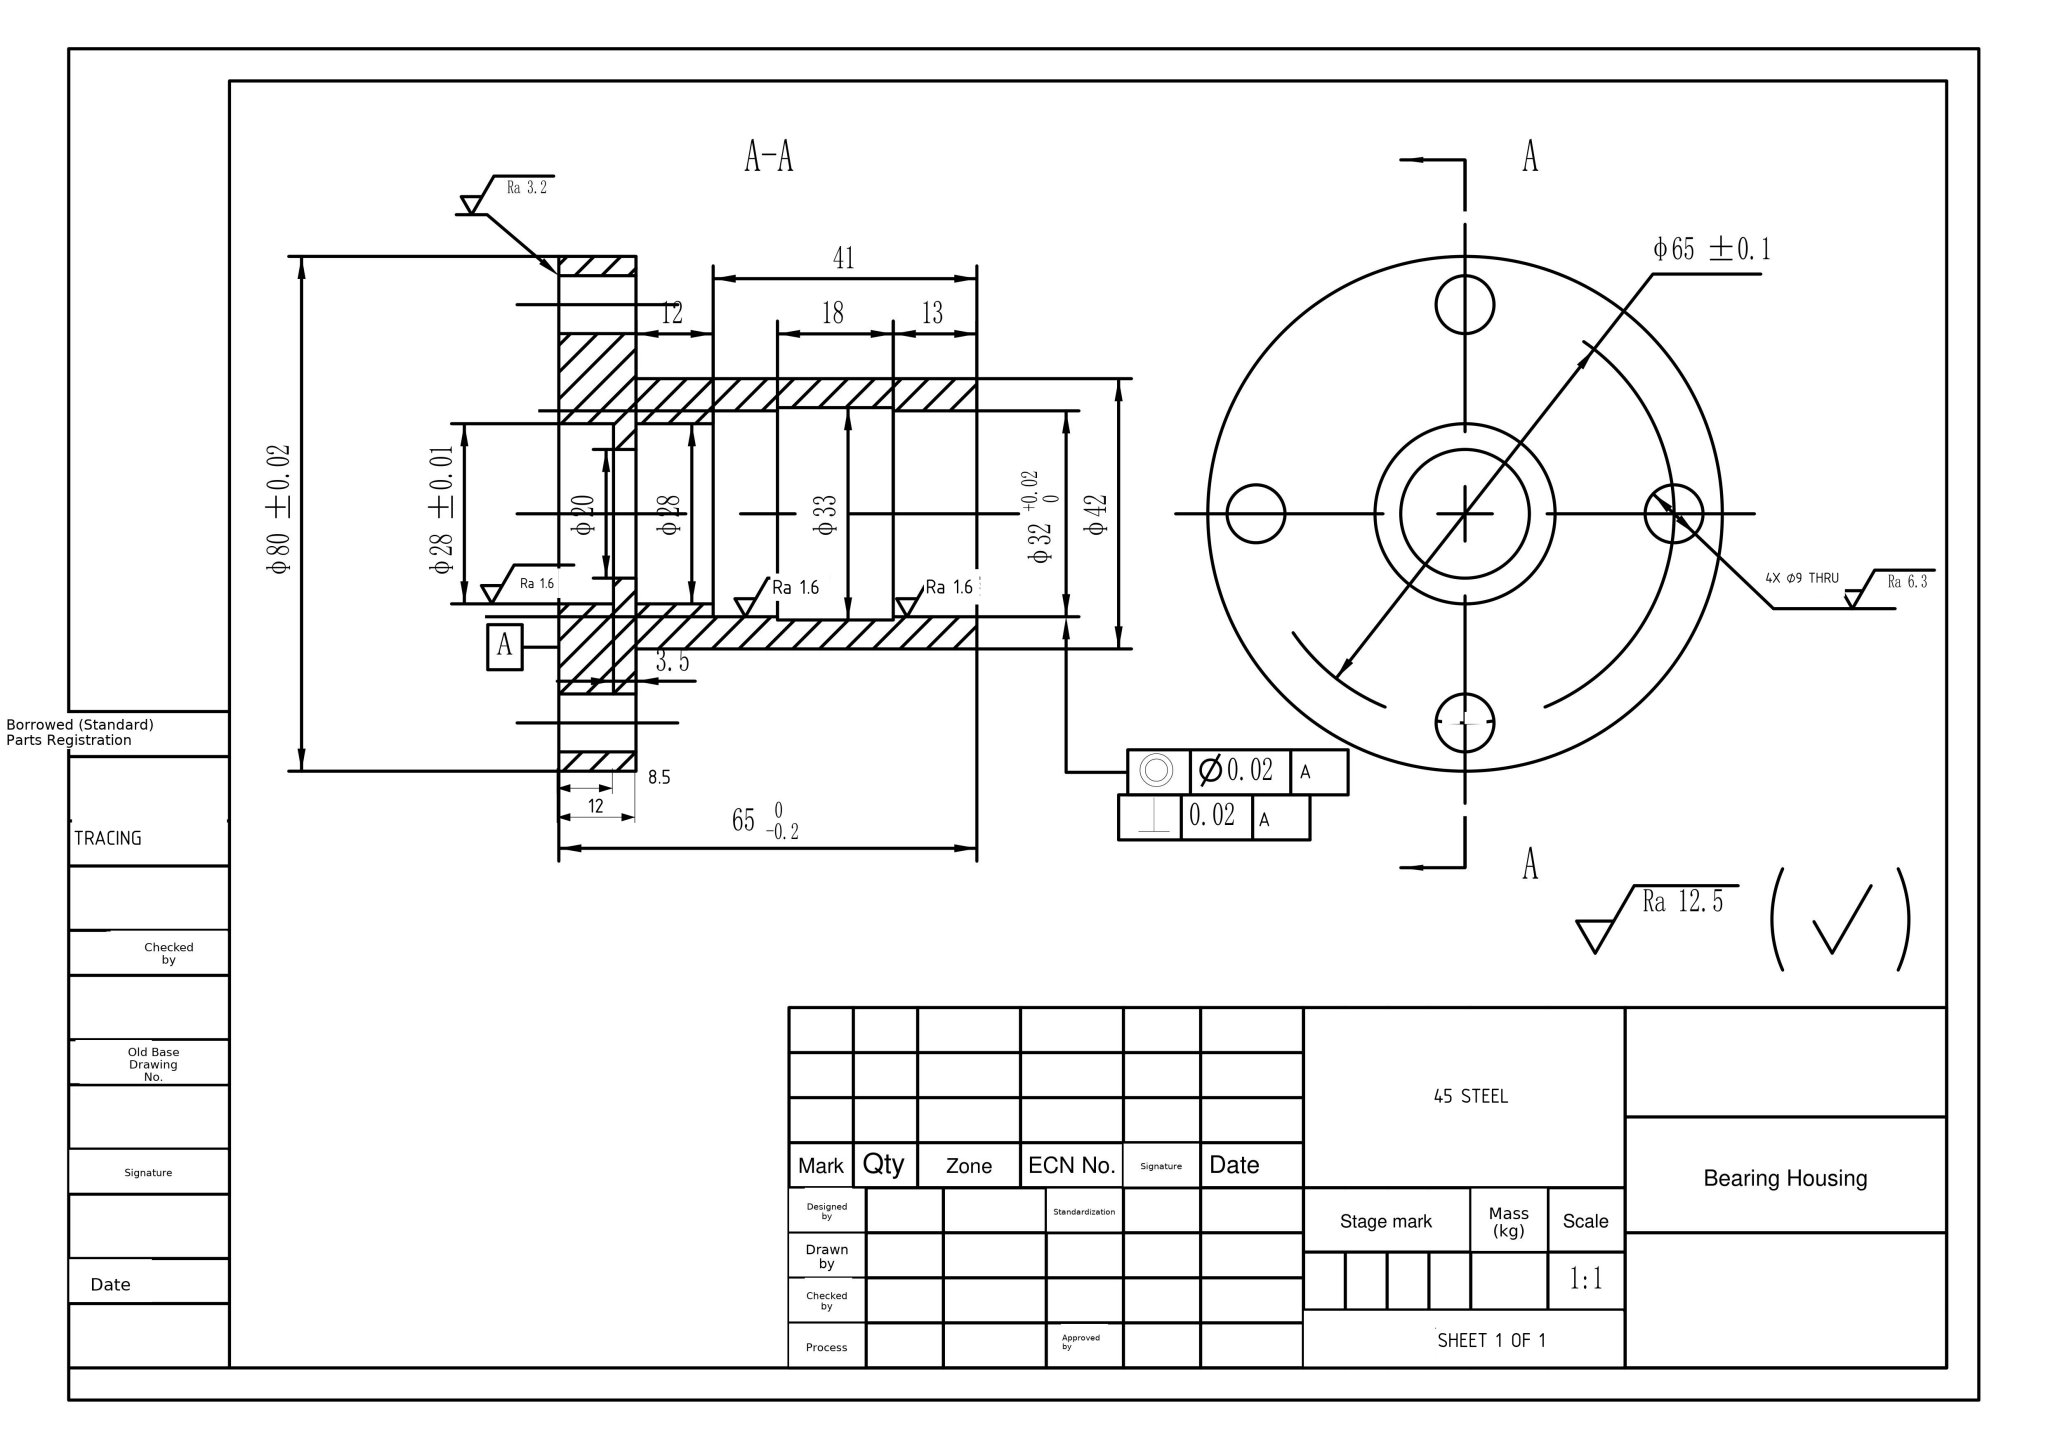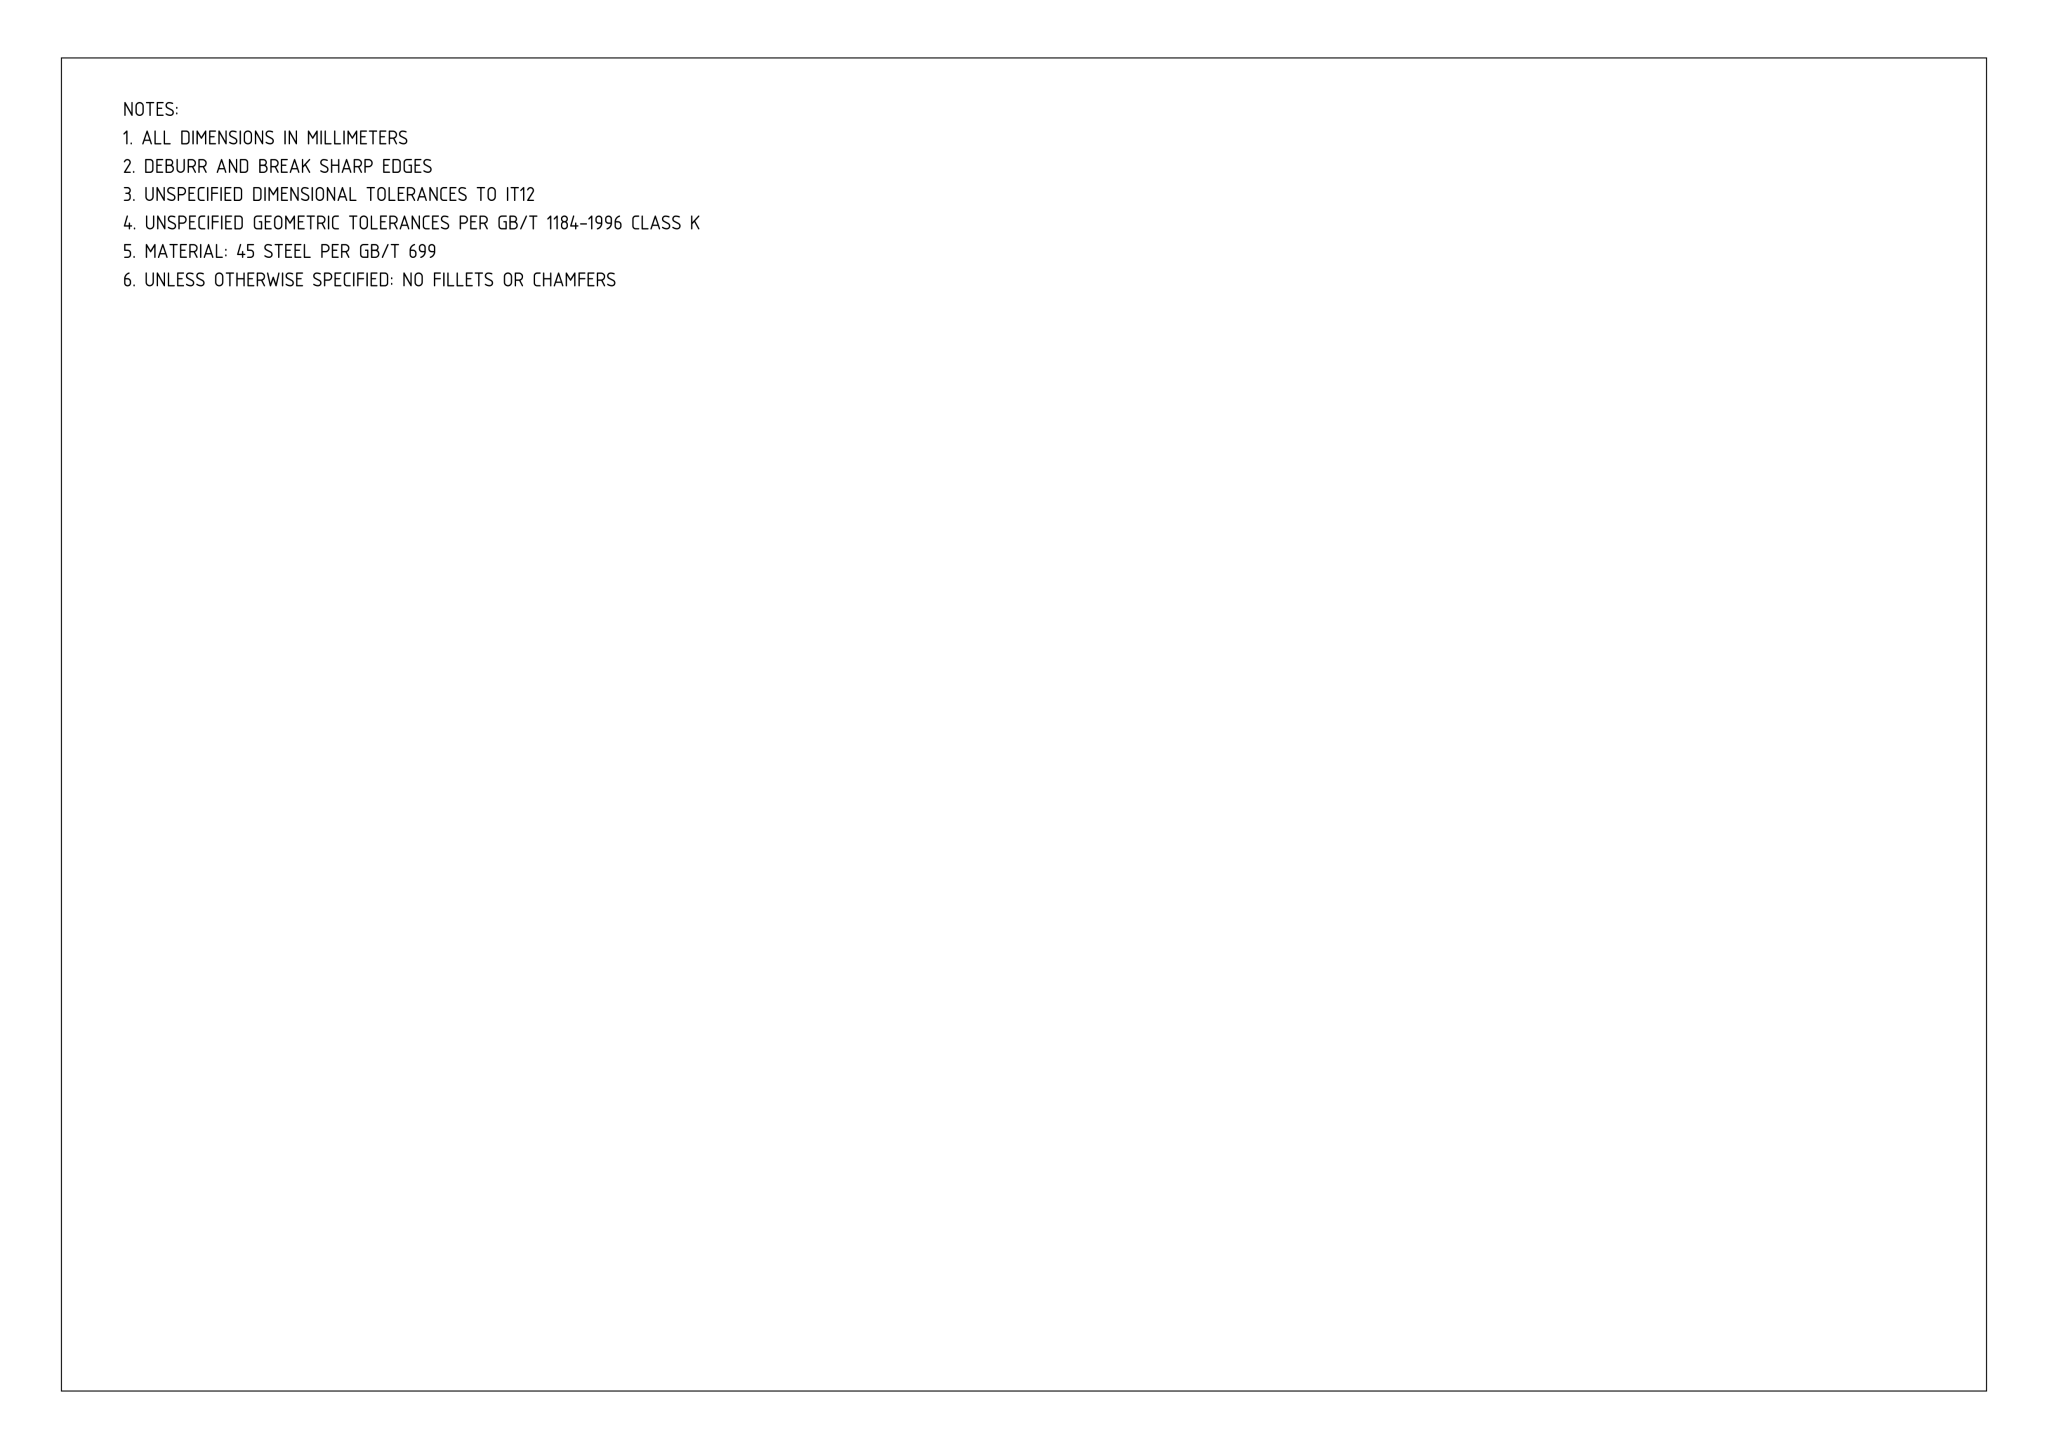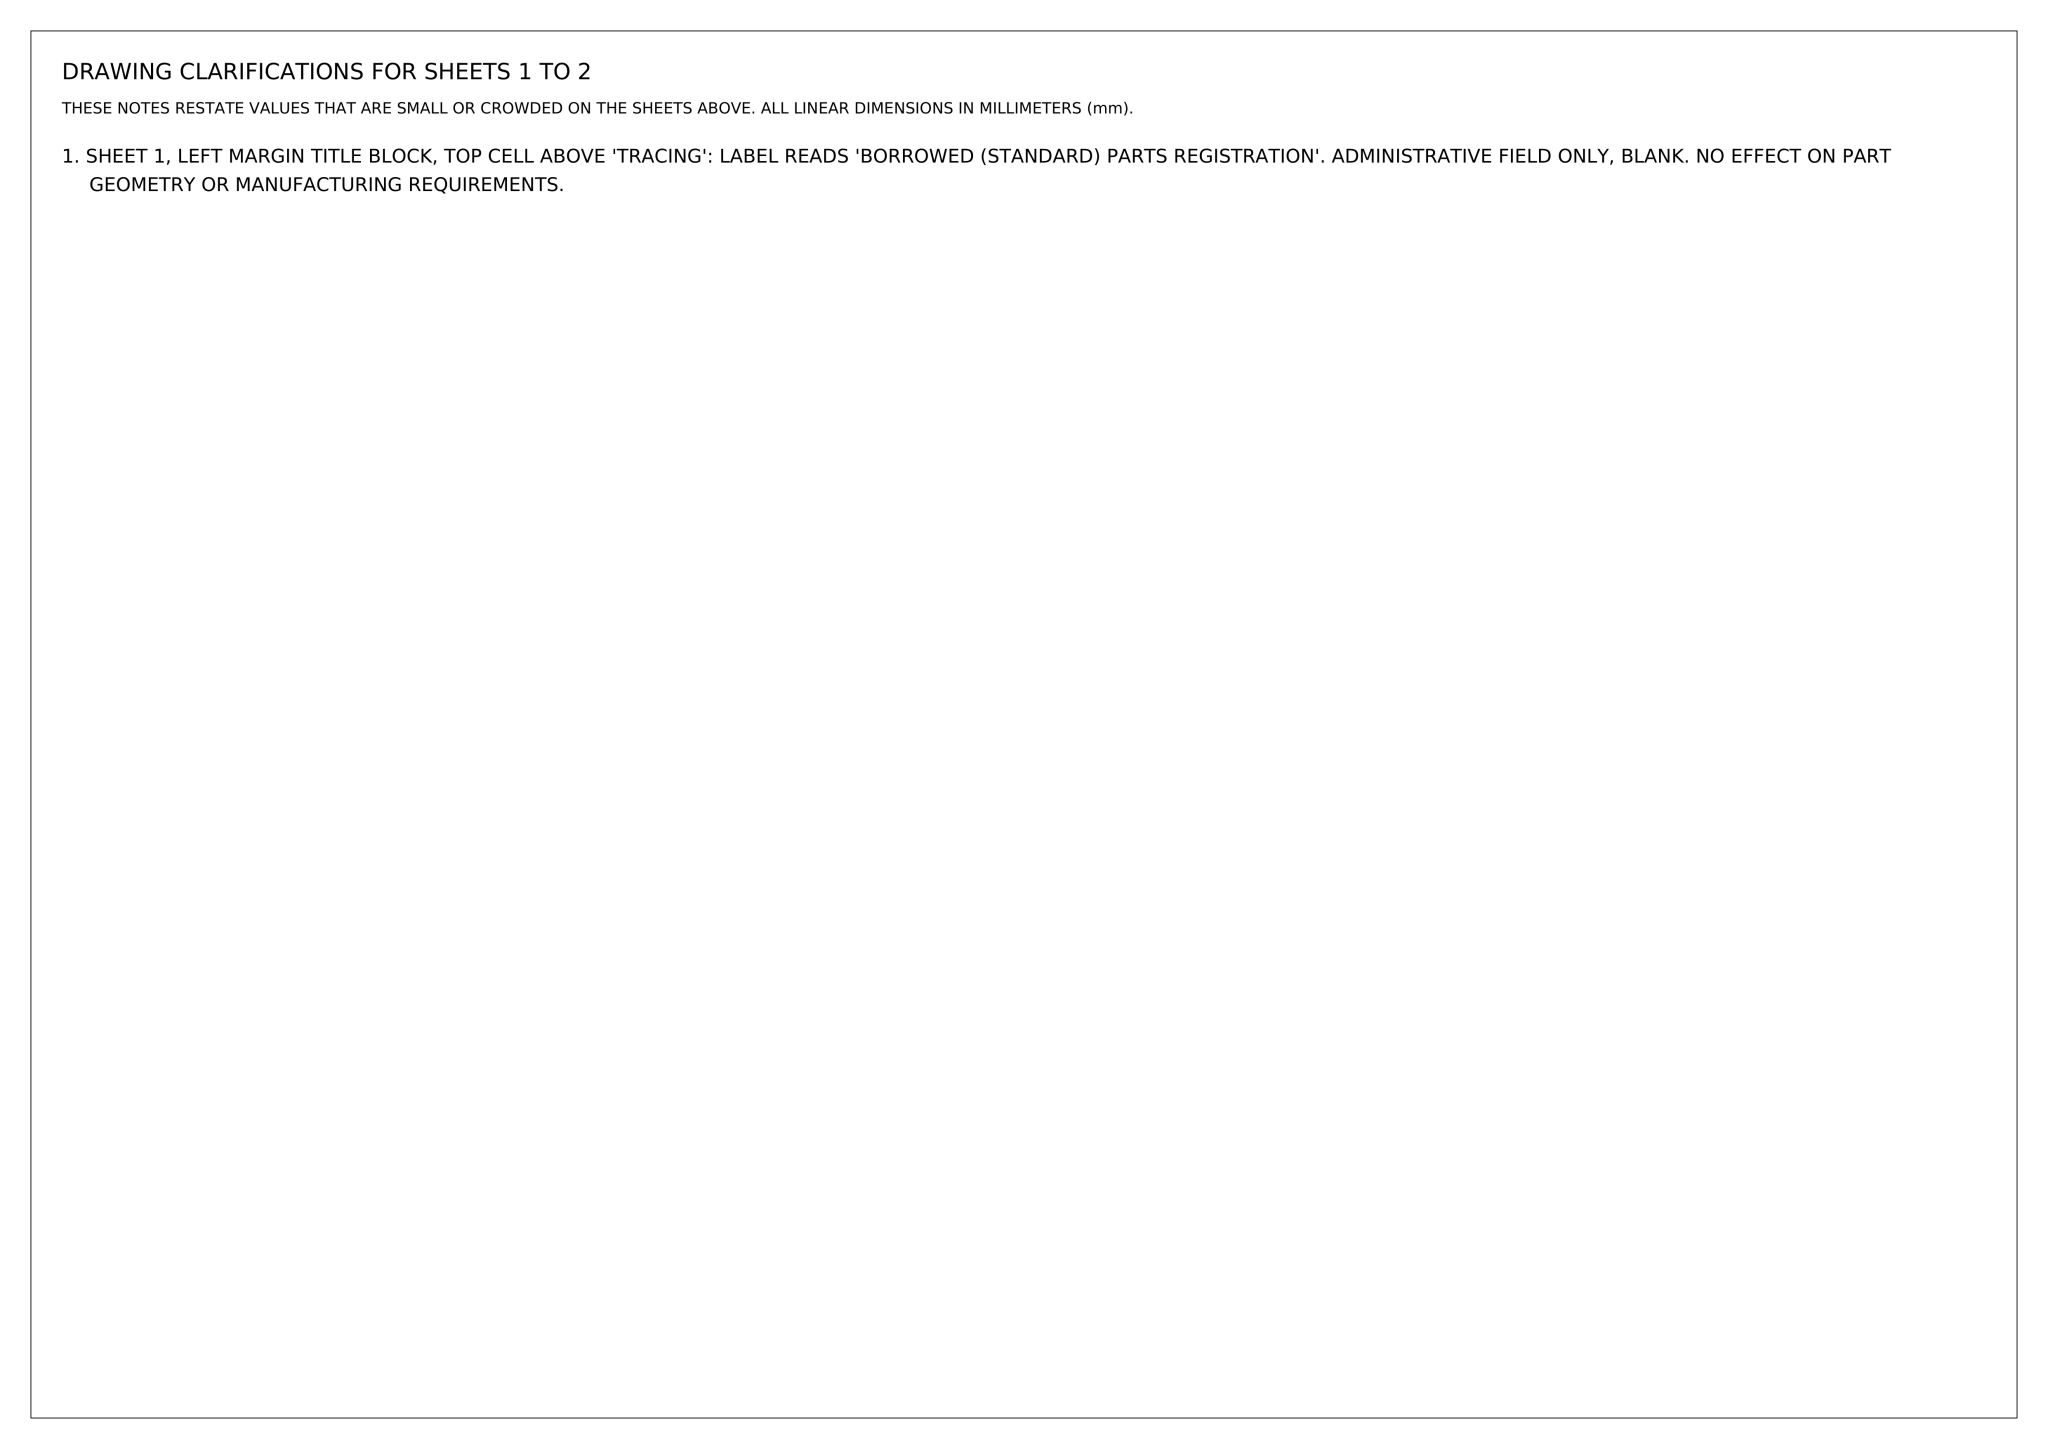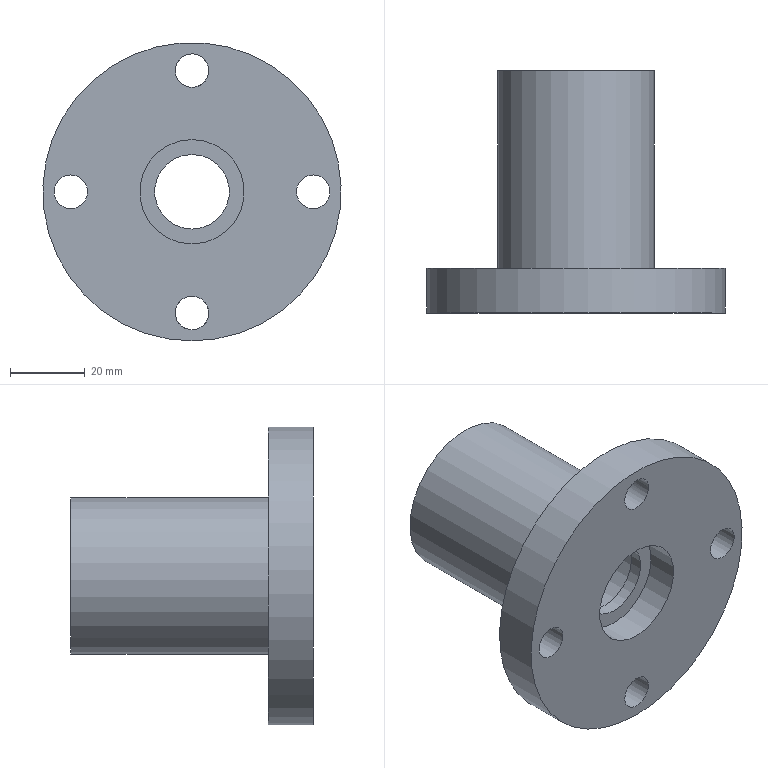Part | NX | mm | 1 solid | 20 faces | box 80 x 65 x 80 mm | volume 83078 mm3 | cylinder 12 | plane 8 | commonest cylinder face diameters 9 x4 28 x2 32 x2 20 x1 33 x1 42 x1 80 x1
STEP:
#1=CARTESIAN_POINT('',(0.,0.,0.));
#2=DIRECTION('',(0.,0.,1.));
#3=DIRECTION('',(1.,0.,0.));
#4=AXIS2_PLACEMENT_3D('',#1,#2,#3);
#5=(LENGTH_UNIT()NAMED_UNIT(*)SI_UNIT(.MILLI.,.METRE.));
#6=UNCERTAINTY_MEASURE_WITH_UNIT(LENGTH_MEASURE(0.00002),#5,'','');
#7=(NAMED_UNIT(*)PLANE_ANGLE_UNIT()SI_UNIT($,.RADIAN.));
#8=PLANE_ANGLE_MEASURE_WITH_UNIT(PLANE_ANGLE_MEASURE(0.01745),#7);
#9=DIMENSIONAL_EXPONENTS(0.,0.,0.,0.,0.,0.,0.);
#10=(CONVERSION_BASED_UNIT('',#8)NAMED_UNIT(#9)PLANE_ANGLE_UNIT());
#11=(NAMED_UNIT(*)SI_UNIT($,.STERADIAN.)SOLID_ANGLE_UNIT());
#12=(GEOMETRIC_REPRESENTATION_CONTEXT(3)GLOBAL_UNCERTAINTY_ASSIGNED_CONTEXT((#6))GLOBAL_UNIT_ASSIGNED_CONTEXT((#5,#10,#11))REPRESENTATION_CONTEXT('',''));
#13=SHAPE_REPRESENTATION('',(#4),#12);
#14=CARTESIAN_POINT('',(32.5,0.,-4.5));
#15=VERTEX_POINT('',#14);
#16=CARTESIAN_POINT('',(32.5,0.,0.));
#17=DIRECTION('',(0.,-1.,0.));
#18=DIRECTION('',(0.,0.,-1.));
#19=AXIS2_PLACEMENT_3D('',#16,#17,#18);
#20=CIRCLE('',#19,4.5);
#21=EDGE_CURVE('',#15,#15,#20,.T.);
#22=ORIENTED_EDGE('',*,*,#21,.F.);
#23=EDGE_LOOP('',(#22));
#24=FACE_BOUND('',#23,.T.);
#25=CARTESIAN_POINT('',(-4.5,0.,-32.5));
#26=VERTEX_POINT('',#25);
#27=CARTESIAN_POINT('',(0.,0.,-32.5));
#28=DIRECTION('',(0.,-1.,0.));
#29=DIRECTION('',(-1.,0.,0.));
#30=AXIS2_PLACEMENT_3D('',#27,#28,#29);
#31=CIRCLE('',#30,4.5);
#32=EDGE_CURVE('',#26,#26,#31,.T.);
#33=ORIENTED_EDGE('',*,*,#32,.F.);
#34=EDGE_LOOP('',(#33));
#35=FACE_BOUND('',#34,.T.);
#36=CARTESIAN_POINT('',(-32.5,0.,4.5));
#37=VERTEX_POINT('',#36);
#38=CARTESIAN_POINT('',(-32.5,0.,0.));
#39=DIRECTION('',(0.,-1.,0.));
#40=DIRECTION('',(0.,0.,1.));
#41=AXIS2_PLACEMENT_3D('',#38,#39,#40);
#42=CIRCLE('',#41,4.5);
#43=EDGE_CURVE('',#37,#37,#42,.T.);
#44=ORIENTED_EDGE('',*,*,#43,.F.);
#45=EDGE_LOOP('',(#44));
#46=FACE_BOUND('',#45,.T.);
#47=CARTESIAN_POINT('',(4.5,0.,32.5));
#48=VERTEX_POINT('',#47);
#49=CARTESIAN_POINT('',(0.,0.,32.5));
#50=DIRECTION('',(0.,-1.,0.));
#51=DIRECTION('',(1.,0.,0.));
#52=AXIS2_PLACEMENT_3D('',#49,#50,#51);
#53=CIRCLE('',#52,4.5);
#54=EDGE_CURVE('',#48,#48,#53,.T.);
#55=ORIENTED_EDGE('',*,*,#54,.F.);
#56=EDGE_LOOP('',(#55));
#57=FACE_BOUND('',#56,.T.);
#58=CARTESIAN_POINT('',(0.,0.,-14.));
#59=VERTEX_POINT('',#58);
#60=CARTESIAN_POINT('',(0.,0.,0.));
#61=DIRECTION('',(0.,-1.,0.));
#62=DIRECTION('',(0.,0.,-1.));
#63=AXIS2_PLACEMENT_3D('',#60,#61,#62);
#64=CIRCLE('',#63,14.);
#65=EDGE_CURVE('',#59,#59,#64,.T.);
#66=ORIENTED_EDGE('',*,*,#65,.F.);
#67=EDGE_LOOP('',(#66));
#68=FACE_BOUND('',#67,.T.);
#69=CARTESIAN_POINT('',(0.,0.,-40.));
#70=VERTEX_POINT('',#69);
#71=CARTESIAN_POINT('',(0.,0.,0.));
#72=DIRECTION('',(0.,-1.,0.));
#73=DIRECTION('',(0.,0.,-1.));
#74=AXIS2_PLACEMENT_3D('',#71,#72,#73);
#75=CIRCLE('',#74,40.);
#76=EDGE_CURVE('',#70,#70,#75,.T.);
#77=ORIENTED_EDGE('',*,*,#76,.T.);
#78=EDGE_LOOP('',(#77));
#79=FACE_BOUND('',#78,.T.);
#80=CARTESIAN_POINT('',(0.,0.,40.));
#81=DIRECTION('',(0.,1.,0.));
#82=DIRECTION('',(0.,0.,1.));
#83=AXIS2_PLACEMENT_3D('',#80,#81,#82);
#84=PLANE('',#83);
#85=ADVANCED_FACE('',(#24,#35,#46,#57,#68,#79),#84,.F.);
#86=CARTESIAN_POINT('',(0.,8.5,-14.));
#87=VERTEX_POINT('',#86);
#88=CARTESIAN_POINT('',(0.,8.5,0.));
#89=DIRECTION('',(0.,-1.,0.));
#90=DIRECTION('',(0.,0.,-1.));
#91=AXIS2_PLACEMENT_3D('',#88,#89,#90);
#92=CIRCLE('',#91,14.);
#93=EDGE_CURVE('',#87,#87,#92,.T.);
#94=ORIENTED_EDGE('',*,*,#93,.F.);
#95=EDGE_LOOP('',(#94));
#96=FACE_BOUND('',#95,.T.);
#97=ORIENTED_EDGE('',*,*,#65,.T.);
#98=EDGE_LOOP('',(#97));
#99=FACE_BOUND('',#98,.T.);
#100=CARTESIAN_POINT('',(0.,0.,0.));
#101=DIRECTION('',(0.,-1.,0.));
#102=DIRECTION('',(0.,0.,-1.));
#103=AXIS2_PLACEMENT_3D('',#100,#101,#102);
#104=CYLINDRICAL_SURFACE('',#103,14.);
#105=ADVANCED_FACE('',(#96,#99),#104,.F.);
#106=CARTESIAN_POINT('',(0.,8.5,-10.));
#107=VERTEX_POINT('',#106);
#108=CARTESIAN_POINT('',(0.,8.5,0.));
#109=DIRECTION('',(0.,-1.,0.));
#110=DIRECTION('',(0.,0.,-1.));
#111=AXIS2_PLACEMENT_3D('',#108,#109,#110);
#112=CIRCLE('',#111,10.);
#113=EDGE_CURVE('',#107,#107,#112,.T.);
#114=ORIENTED_EDGE('',*,*,#113,.F.);
#115=EDGE_LOOP('',(#114));
#116=FACE_BOUND('',#115,.T.);
#117=ORIENTED_EDGE('',*,*,#93,.T.);
#118=EDGE_LOOP('',(#117));
#119=FACE_BOUND('',#118,.T.);
#120=CARTESIAN_POINT('',(0.,8.5,14.));
#121=DIRECTION('',(0.,1.,0.));
#122=DIRECTION('',(0.,0.,1.));
#123=AXIS2_PLACEMENT_3D('',#120,#121,#122);
#124=PLANE('',#123);
#125=ADVANCED_FACE('',(#116,#119),#124,.F.);
#126=CARTESIAN_POINT('',(0.,12.,-10.));
#127=VERTEX_POINT('',#126);
#128=CARTESIAN_POINT('',(0.,12.,0.));
#129=DIRECTION('',(0.,-1.,0.));
#130=DIRECTION('',(0.,0.,-1.));
#131=AXIS2_PLACEMENT_3D('',#128,#129,#130);
#132=CIRCLE('',#131,10.);
#133=EDGE_CURVE('',#127,#127,#132,.T.);
#134=ORIENTED_EDGE('',*,*,#133,.F.);
#135=EDGE_LOOP('',(#134));
#136=FACE_BOUND('',#135,.T.);
#137=ORIENTED_EDGE('',*,*,#113,.T.);
#138=EDGE_LOOP('',(#137));
#139=FACE_BOUND('',#138,.T.);
#140=CARTESIAN_POINT('',(0.,0.,0.));
#141=DIRECTION('',(0.,-1.,0.));
#142=DIRECTION('',(0.,0.,-1.));
#143=AXIS2_PLACEMENT_3D('',#140,#141,#142);
#144=CYLINDRICAL_SURFACE('',#143,10.);
#145=ADVANCED_FACE('',(#136,#139),#144,.F.);
#146=CARTESIAN_POINT('',(0.,12.,-14.));
#147=VERTEX_POINT('',#146);
#148=CARTESIAN_POINT('',(0.,12.,0.));
#149=DIRECTION('',(0.,-1.,0.));
#150=DIRECTION('',(0.,0.,-1.));
#151=AXIS2_PLACEMENT_3D('',#148,#149,#150);
#152=CIRCLE('',#151,14.);
#153=EDGE_CURVE('',#147,#147,#152,.T.);
#154=ORIENTED_EDGE('',*,*,#153,.F.);
#155=EDGE_LOOP('',(#154));
#156=FACE_BOUND('',#155,.T.);
#157=ORIENTED_EDGE('',*,*,#133,.T.);
#158=EDGE_LOOP('',(#157));
#159=FACE_BOUND('',#158,.T.);
#160=CARTESIAN_POINT('',(0.,12.,10.));
#161=DIRECTION('',(0.,-1.,0.));
#162=DIRECTION('',(0.,0.,-1.));
#163=AXIS2_PLACEMENT_3D('',#160,#161,#162);
#164=PLANE('',#163);
#165=ADVANCED_FACE('',(#156,#159),#164,.F.);
#166=CARTESIAN_POINT('',(0.,24.,-14.));
#167=VERTEX_POINT('',#166);
#168=CARTESIAN_POINT('',(0.,24.,0.));
#169=DIRECTION('',(0.,-1.,0.));
#170=DIRECTION('',(0.,0.,-1.));
#171=AXIS2_PLACEMENT_3D('',#168,#169,#170);
#172=CIRCLE('',#171,14.);
#173=EDGE_CURVE('',#167,#167,#172,.T.);
#174=ORIENTED_EDGE('',*,*,#173,.F.);
#175=EDGE_LOOP('',(#174));
#176=FACE_BOUND('',#175,.T.);
#177=ORIENTED_EDGE('',*,*,#153,.T.);
#178=EDGE_LOOP('',(#177));
#179=FACE_BOUND('',#178,.T.);
#180=CARTESIAN_POINT('',(0.,0.,0.));
#181=DIRECTION('',(0.,-1.,0.));
#182=DIRECTION('',(0.,0.,-1.));
#183=AXIS2_PLACEMENT_3D('',#180,#181,#182);
#184=CYLINDRICAL_SURFACE('',#183,14.);
#185=ADVANCED_FACE('',(#176,#179),#184,.F.);
#186=CARTESIAN_POINT('',(0.,24.,-16.));
#187=VERTEX_POINT('',#186);
#188=CARTESIAN_POINT('',(0.,24.,0.));
#189=DIRECTION('',(0.,-1.,0.));
#190=DIRECTION('',(0.,0.,-1.));
#191=AXIS2_PLACEMENT_3D('',#188,#189,#190);
#192=CIRCLE('',#191,16.);
#193=EDGE_CURVE('',#187,#187,#192,.T.);
#194=ORIENTED_EDGE('',*,*,#193,.F.);
#195=EDGE_LOOP('',(#194));
#196=FACE_BOUND('',#195,.T.);
#197=ORIENTED_EDGE('',*,*,#173,.T.);
#198=EDGE_LOOP('',(#197));
#199=FACE_BOUND('',#198,.T.);
#200=CARTESIAN_POINT('',(0.,24.,14.));
#201=DIRECTION('',(0.,-1.,0.));
#202=DIRECTION('',(0.,0.,-1.));
#203=AXIS2_PLACEMENT_3D('',#200,#201,#202);
#204=PLANE('',#203);
#205=ADVANCED_FACE('',(#196,#199),#204,.F.);
#206=CARTESIAN_POINT('',(0.,34.,-16.));
#207=VERTEX_POINT('',#206);
#208=CARTESIAN_POINT('',(0.,34.,0.));
#209=DIRECTION('',(0.,-1.,0.));
#210=DIRECTION('',(0.,0.,-1.));
#211=AXIS2_PLACEMENT_3D('',#208,#209,#210);
#212=CIRCLE('',#211,16.);
#213=EDGE_CURVE('',#207,#207,#212,.T.);
#214=ORIENTED_EDGE('',*,*,#213,.F.);
#215=EDGE_LOOP('',(#214));
#216=FACE_BOUND('',#215,.T.);
#217=ORIENTED_EDGE('',*,*,#193,.T.);
#218=EDGE_LOOP('',(#217));
#219=FACE_BOUND('',#218,.T.);
#220=CARTESIAN_POINT('',(0.,0.,0.));
#221=DIRECTION('',(0.,-1.,0.));
#222=DIRECTION('',(0.,0.,-1.));
#223=AXIS2_PLACEMENT_3D('',#220,#221,#222);
#224=CYLINDRICAL_SURFACE('',#223,16.);
#225=ADVANCED_FACE('',(#216,#219),#224,.F.);
#226=CARTESIAN_POINT('',(0.,34.,-16.5));
#227=VERTEX_POINT('',#226);
#228=CARTESIAN_POINT('',(0.,34.,0.));
#229=DIRECTION('',(0.,-1.,0.));
#230=DIRECTION('',(0.,0.,-1.));
#231=AXIS2_PLACEMENT_3D('',#228,#229,#230);
#232=CIRCLE('',#231,16.5);
#233=EDGE_CURVE('',#227,#227,#232,.T.);
#234=ORIENTED_EDGE('',*,*,#233,.F.);
#235=EDGE_LOOP('',(#234));
#236=FACE_BOUND('',#235,.T.);
#237=ORIENTED_EDGE('',*,*,#213,.T.);
#238=EDGE_LOOP('',(#237));
#239=FACE_BOUND('',#238,.T.);
#240=CARTESIAN_POINT('',(0.,34.,16.));
#241=DIRECTION('',(0.,-1.,0.));
#242=DIRECTION('',(0.,0.,-1.));
#243=AXIS2_PLACEMENT_3D('',#240,#241,#242);
#244=PLANE('',#243);
#245=ADVANCED_FACE('',(#236,#239),#244,.F.);
#246=CARTESIAN_POINT('',(0.,52.,-16.5));
#247=VERTEX_POINT('',#246);
#248=CARTESIAN_POINT('',(0.,52.,0.));
#249=DIRECTION('',(0.,-1.,0.));
#250=DIRECTION('',(0.,0.,-1.));
#251=AXIS2_PLACEMENT_3D('',#248,#249,#250);
#252=CIRCLE('',#251,16.5);
#253=EDGE_CURVE('',#247,#247,#252,.T.);
#254=ORIENTED_EDGE('',*,*,#253,.F.);
#255=EDGE_LOOP('',(#254));
#256=FACE_BOUND('',#255,.T.);
#257=ORIENTED_EDGE('',*,*,#233,.T.);
#258=EDGE_LOOP('',(#257));
#259=FACE_BOUND('',#258,.T.);
#260=CARTESIAN_POINT('',(0.,0.,0.));
#261=DIRECTION('',(0.,-1.,0.));
#262=DIRECTION('',(0.,0.,-1.));
#263=AXIS2_PLACEMENT_3D('',#260,#261,#262);
#264=CYLINDRICAL_SURFACE('',#263,16.5);
#265=ADVANCED_FACE('',(#256,#259),#264,.F.);
#266=CARTESIAN_POINT('',(0.,52.,-16.));
#267=VERTEX_POINT('',#266);
#268=CARTESIAN_POINT('',(0.,52.,0.));
#269=DIRECTION('',(0.,-1.,0.));
#270=DIRECTION('',(0.,0.,-1.));
#271=AXIS2_PLACEMENT_3D('',#268,#269,#270);
#272=CIRCLE('',#271,16.);
#273=EDGE_CURVE('',#267,#267,#272,.T.);
#274=ORIENTED_EDGE('',*,*,#273,.F.);
#275=EDGE_LOOP('',(#274));
#276=FACE_BOUND('',#275,.T.);
#277=ORIENTED_EDGE('',*,*,#253,.T.);
#278=EDGE_LOOP('',(#277));
#279=FACE_BOUND('',#278,.T.);
#280=CARTESIAN_POINT('',(0.,52.,16.5));
#281=DIRECTION('',(0.,1.,0.));
#282=DIRECTION('',(0.,0.,1.));
#283=AXIS2_PLACEMENT_3D('',#280,#281,#282);
#284=PLANE('',#283);
#285=ADVANCED_FACE('',(#276,#279),#284,.F.);
#286=CARTESIAN_POINT('',(0.,65.,-16.));
#287=VERTEX_POINT('',#286);
#288=CARTESIAN_POINT('',(0.,65.,0.));
#289=DIRECTION('',(0.,-1.,0.));
#290=DIRECTION('',(0.,0.,-1.));
#291=AXIS2_PLACEMENT_3D('',#288,#289,#290);
#292=CIRCLE('',#291,16.);
#293=EDGE_CURVE('',#287,#287,#292,.T.);
#294=ORIENTED_EDGE('',*,*,#293,.F.);
#295=EDGE_LOOP('',(#294));
#296=FACE_BOUND('',#295,.T.);
#297=ORIENTED_EDGE('',*,*,#273,.T.);
#298=EDGE_LOOP('',(#297));
#299=FACE_BOUND('',#298,.T.);
#300=CARTESIAN_POINT('',(0.,0.,0.));
#301=DIRECTION('',(0.,-1.,0.));
#302=DIRECTION('',(0.,0.,-1.));
#303=AXIS2_PLACEMENT_3D('',#300,#301,#302);
#304=CYLINDRICAL_SURFACE('',#303,16.);
#305=ADVANCED_FACE('',(#296,#299),#304,.F.);
#306=CARTESIAN_POINT('',(0.,65.,-21.));
#307=VERTEX_POINT('',#306);
#308=CARTESIAN_POINT('',(0.,65.,0.));
#309=DIRECTION('',(0.,-1.,0.));
#310=DIRECTION('',(0.,0.,-1.));
#311=AXIS2_PLACEMENT_3D('',#308,#309,#310);
#312=CIRCLE('',#311,21.);
#313=EDGE_CURVE('',#307,#307,#312,.T.);
#314=ORIENTED_EDGE('',*,*,#313,.F.);
#315=EDGE_LOOP('',(#314));
#316=FACE_BOUND('',#315,.T.);
#317=ORIENTED_EDGE('',*,*,#293,.T.);
#318=EDGE_LOOP('',(#317));
#319=FACE_BOUND('',#318,.T.);
#320=CARTESIAN_POINT('',(0.,65.,16.));
#321=DIRECTION('',(0.,-1.,0.));
#322=DIRECTION('',(0.,0.,-1.));
#323=AXIS2_PLACEMENT_3D('',#320,#321,#322);
#324=PLANE('',#323);
#325=ADVANCED_FACE('',(#316,#319),#324,.F.);
#326=CARTESIAN_POINT('',(0.,12.,-21.));
#327=VERTEX_POINT('',#326);
#328=CARTESIAN_POINT('',(0.,12.,0.));
#329=DIRECTION('',(0.,-1.,0.));
#330=DIRECTION('',(0.,0.,-1.));
#331=AXIS2_PLACEMENT_3D('',#328,#329,#330);
#332=CIRCLE('',#331,21.);
#333=EDGE_CURVE('',#327,#327,#332,.T.);
#334=ORIENTED_EDGE('',*,*,#333,.F.);
#335=EDGE_LOOP('',(#334));
#336=FACE_BOUND('',#335,.T.);
#337=ORIENTED_EDGE('',*,*,#313,.T.);
#338=EDGE_LOOP('',(#337));
#339=FACE_BOUND('',#338,.T.);
#340=CARTESIAN_POINT('',(0.,0.,0.));
#341=DIRECTION('',(0.,-1.,0.));
#342=DIRECTION('',(0.,0.,-1.));
#343=AXIS2_PLACEMENT_3D('',#340,#341,#342);
#344=CYLINDRICAL_SURFACE('',#343,21.);
#345=ADVANCED_FACE('',(#336,#339),#344,.T.);
#346=CARTESIAN_POINT('',(32.5,12.,-4.5));
#347=VERTEX_POINT('',#346);
#348=CARTESIAN_POINT('',(32.5,12.,0.));
#349=DIRECTION('',(0.,-1.,0.));
#350=DIRECTION('',(0.,0.,-1.));
#351=AXIS2_PLACEMENT_3D('',#348,#349,#350);
#352=CIRCLE('',#351,4.5);
#353=EDGE_CURVE('',#347,#347,#352,.T.);
#354=ORIENTED_EDGE('',*,*,#353,.T.);
#355=EDGE_LOOP('',(#354));
#356=FACE_BOUND('',#355,.T.);
#357=CARTESIAN_POINT('',(0.,12.,-37.));
#358=VERTEX_POINT('',#357);
#359=CARTESIAN_POINT('',(0.,12.,-32.5));
#360=DIRECTION('',(0.,-1.,0.));
#361=DIRECTION('',(0.,0.,-1.));
#362=AXIS2_PLACEMENT_3D('',#359,#360,#361);
#363=CIRCLE('',#362,4.5);
#364=EDGE_CURVE('',#358,#358,#363,.T.);
#365=ORIENTED_EDGE('',*,*,#364,.T.);
#366=EDGE_LOOP('',(#365));
#367=FACE_BOUND('',#366,.T.);
#368=CARTESIAN_POINT('',(-32.5,12.,-4.5));
#369=VERTEX_POINT('',#368);
#370=CARTESIAN_POINT('',(-32.5,12.,0.));
#371=DIRECTION('',(0.,-1.,0.));
#372=DIRECTION('',(0.,0.,-1.));
#373=AXIS2_PLACEMENT_3D('',#370,#371,#372);
#374=CIRCLE('',#373,4.5);
#375=EDGE_CURVE('',#369,#369,#374,.T.);
#376=ORIENTED_EDGE('',*,*,#375,.T.);
#377=EDGE_LOOP('',(#376));
#378=FACE_BOUND('',#377,.T.);
#379=CARTESIAN_POINT('',(0.,12.,28.));
#380=VERTEX_POINT('',#379);
#381=CARTESIAN_POINT('',(0.,12.,32.5));
#382=DIRECTION('',(0.,-1.,0.));
#383=DIRECTION('',(0.,0.,-1.));
#384=AXIS2_PLACEMENT_3D('',#381,#382,#383);
#385=CIRCLE('',#384,4.5);
#386=EDGE_CURVE('',#380,#380,#385,.T.);
#387=ORIENTED_EDGE('',*,*,#386,.T.);
#388=EDGE_LOOP('',(#387));
#389=FACE_BOUND('',#388,.T.);
#390=CARTESIAN_POINT('',(0.,12.,-40.));
#391=VERTEX_POINT('',#390);
#392=CARTESIAN_POINT('',(0.,12.,0.));
#393=DIRECTION('',(0.,-1.,0.));
#394=DIRECTION('',(0.,0.,-1.));
#395=AXIS2_PLACEMENT_3D('',#392,#393,#394);
#396=CIRCLE('',#395,40.);
#397=EDGE_CURVE('',#391,#391,#396,.T.);
#398=ORIENTED_EDGE('',*,*,#397,.F.);
#399=EDGE_LOOP('',(#398));
#400=FACE_BOUND('',#399,.T.);
#401=ORIENTED_EDGE('',*,*,#333,.T.);
#402=EDGE_LOOP('',(#401));
#403=FACE_BOUND('',#402,.T.);
#404=CARTESIAN_POINT('',(0.,12.,21.));
#405=DIRECTION('',(0.,-1.,0.));
#406=DIRECTION('',(0.,0.,-1.));
#407=AXIS2_PLACEMENT_3D('',#404,#405,#406);
#408=PLANE('',#407);
#409=ADVANCED_FACE('',(#356,#367,#378,#389,#400,#403),#408,.F.);
#410=ORIENTED_EDGE('',*,*,#76,.F.);
#411=EDGE_LOOP('',(#410));
#412=FACE_BOUND('',#411,.T.);
#413=ORIENTED_EDGE('',*,*,#397,.T.);
#414=EDGE_LOOP('',(#413));
#415=FACE_BOUND('',#414,.T.);
#416=CARTESIAN_POINT('',(0.,0.,0.));
#417=DIRECTION('',(0.,-1.,0.));
#418=DIRECTION('',(0.,0.,-1.));
#419=AXIS2_PLACEMENT_3D('',#416,#417,#418);
#420=CYLINDRICAL_SURFACE('',#419,40.);
#421=ADVANCED_FACE('',(#412,#415),#420,.T.);
#422=ORIENTED_EDGE('',*,*,#54,.T.);
#423=EDGE_LOOP('',(#422));
#424=FACE_BOUND('',#423,.T.);
#425=ORIENTED_EDGE('',*,*,#386,.F.);
#426=EDGE_LOOP('',(#425));
#427=FACE_BOUND('',#426,.T.);
#428=CARTESIAN_POINT('',(0.,50.,32.5));
#429=DIRECTION('',(0.,-1.,0.));
#430=DIRECTION('',(0.,0.,-1.));
#431=AXIS2_PLACEMENT_3D('',#428,#429,#430);
#432=CYLINDRICAL_SURFACE('',#431,4.5);
#433=ADVANCED_FACE('',(#424,#427),#432,.F.);
#434=ORIENTED_EDGE('',*,*,#43,.T.);
#435=EDGE_LOOP('',(#434));
#436=FACE_BOUND('',#435,.T.);
#437=ORIENTED_EDGE('',*,*,#375,.F.);
#438=EDGE_LOOP('',(#437));
#439=FACE_BOUND('',#438,.T.);
#440=CARTESIAN_POINT('',(-32.5,50.,0.));
#441=DIRECTION('',(0.,-1.,0.));
#442=DIRECTION('',(0.,0.,-1.));
#443=AXIS2_PLACEMENT_3D('',#440,#441,#442);
#444=CYLINDRICAL_SURFACE('',#443,4.5);
#445=ADVANCED_FACE('',(#436,#439),#444,.F.);
#446=ORIENTED_EDGE('',*,*,#32,.T.);
#447=EDGE_LOOP('',(#446));
#448=FACE_BOUND('',#447,.T.);
#449=ORIENTED_EDGE('',*,*,#364,.F.);
#450=EDGE_LOOP('',(#449));
#451=FACE_BOUND('',#450,.T.);
#452=CARTESIAN_POINT('',(0.,50.,-32.5));
#453=DIRECTION('',(0.,-1.,0.));
#454=DIRECTION('',(0.,0.,-1.));
#455=AXIS2_PLACEMENT_3D('',#452,#453,#454);
#456=CYLINDRICAL_SURFACE('',#455,4.5);
#457=ADVANCED_FACE('',(#448,#451),#456,.F.);
#458=ORIENTED_EDGE('',*,*,#21,.T.);
#459=EDGE_LOOP('',(#458));
#460=FACE_BOUND('',#459,.T.);
#461=ORIENTED_EDGE('',*,*,#353,.F.);
#462=EDGE_LOOP('',(#461));
#463=FACE_BOUND('',#462,.T.);
#464=CARTESIAN_POINT('',(32.5,50.,0.));
#465=DIRECTION('',(0.,-1.,0.));
#466=DIRECTION('',(0.,0.,-1.));
#467=AXIS2_PLACEMENT_3D('',#464,#465,#466);
#468=CYLINDRICAL_SURFACE('',#467,4.5);
#469=ADVANCED_FACE('',(#460,#463),#468,.F.);
#470=CLOSED_SHELL('',(#85,#105,#125,#145,#165,#185,#205,#225,#245,#265,#285,#305,#325,#345,#409,#421,#433,#445,#457,#469));
#471=MANIFOLD_SOLID_BREP('',#470);
#472=ADVANCED_BREP_SHAPE_REPRESENTATION('',(#471),#12);
#473=SHAPE_REPRESENTATION_RELATIONSHIP('','',#13,#472);
#474=PRESENTATION_LAYER_ASSIGNMENT('','',(#471));
#475=COLOUR_RGB('',1.,0.6,0.);
#476=FILL_AREA_STYLE_COLOUR('',#475);
#477=FILL_AREA_STYLE('',(#476));
#478=SURFACE_STYLE_FILL_AREA(#477);
#479=SURFACE_SIDE_STYLE('',(#478));
#480=SURFACE_STYLE_USAGE(.BOTH.,#479);
#481=PRESENTATION_STYLE_ASSIGNMENT((#480));
#482=STYLED_ITEM('',(#481),#471);
#483=MECHANICAL_DESIGN_GEOMETRIC_PRESENTATION_REPRESENTATION('',(#482),#12);